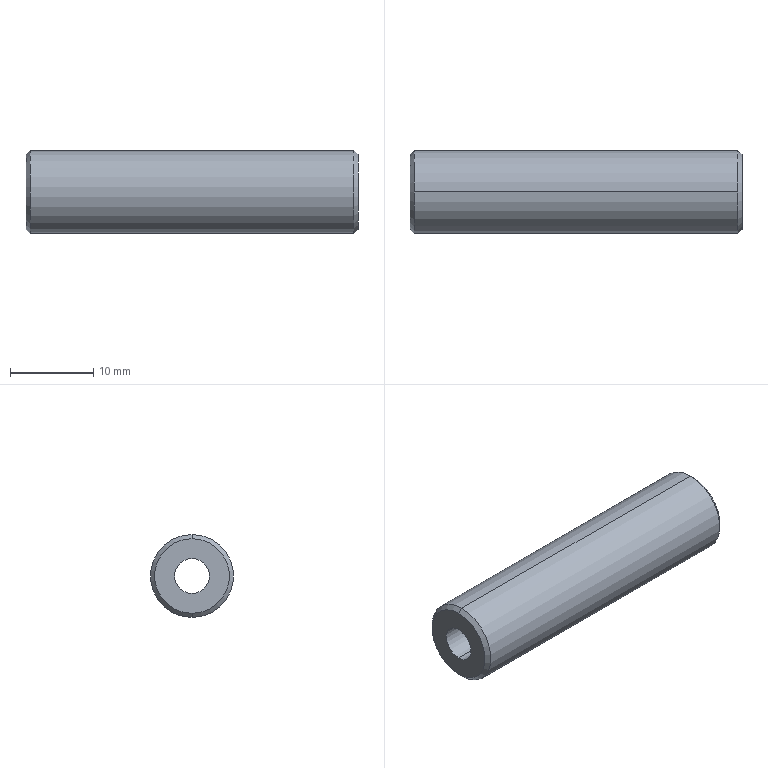Component | SolidWorks | CHEN123-AA-15-2 | 1 solid | 10 faces | box 40 x 10 x 10 mm | volume 2580 mm3 | cone 4 | cylinder 4 | plane 2 | commonest cylinder face diameters 4.2 x2 10 x2
build123d program:
from build123d import *

# Parameters (mm, degrees)
SKETCH1_R           = 5
BOSS_EXTRUDE1_DEPTH = 40
M5_TAPPED_HOLE1_D   = 4.2
CHAMFER1_SIZE       = 0.5


with BuildPart() as part:
    # Sketch1 → Boss-Extrude1 (new body)
    with BuildSketch(Plane.XY):
        Circle(SKETCH1_R)
    extrude(amount=BOSS_EXTRUDE1_DEPTH)

    # M5 Tapped Hole1 (through all)
    with Locations(Plane.XY.offset(40)):
        with Locations((0, 0)):
            Hole(M5_TAPPED_HOLE1_D / 2)

    # Chamfer1
    chamfer1_edges = [part.edges().sort_by_distance(p)[0] for p in [
        (-5, 0, 0),
        (-5, 0, 40),
    ]]
    chamfer(chamfer1_edges, length=CHAMFER1_SIZE)


solid = part.part

# Placed as in the assembly
solid = solid.moved(Location((-20, -132.097, -158.067), (0, 90, 0)))
STEP:
#1=COLOUR_RGB('',0.7922,0.8196,0.9333);
#2=FILL_AREA_STYLE_COLOUR('',#1);
#3=FILL_AREA_STYLE('',(#2));
#4=SURFACE_STYLE_FILL_AREA(#3);
#5=SURFACE_SIDE_STYLE('',(#4));
#6=SURFACE_STYLE_USAGE(.BOTH.,#5);
#7=PRESENTATION_STYLE_ASSIGNMENT((#6));
#8=CARTESIAN_POINT('',(-0.7874,-5.201,-6.046));
#9=VERTEX_POINT('',#8);
#10=CARTESIAN_POINT('',(-0.7874,-5.201,-6.4));
#11=VERTEX_POINT('',#10);
#12=CARTESIAN_POINT('',(-0.7874,-5.201,-6.223));
#13=DIRECTION('',(-1.,0.,0.));
#14=DIRECTION('',(0.,0.,1.));
#15=AXIS2_PLACEMENT_3D('',#12,#13,#14);
#16=CIRCLE('',#15,0.1772);
#17=EDGE_CURVE('',#9,#11,#16,.T.);
#18=ORIENTED_EDGE('',*,*,#17,.F.);
#19=CARTESIAN_POINT('',(-0.7677,-5.201,-6.026));
#20=VERTEX_POINT('',#19);
#21=CARTESIAN_POINT('',(-0.7874,-5.201,-6.046));
#22=DIRECTION('',(0.7071,0.,0.7071));
#23=VECTOR('',#22,39.37);
#24=LINE('',#21,#23);
#25=EDGE_CURVE('',#9,#20,#24,.T.);
#26=ORIENTED_EDGE('',*,*,#25,.T.);
#27=CARTESIAN_POINT('',(-0.7677,-5.201,-6.42));
#28=VERTEX_POINT('',#27);
#29=CARTESIAN_POINT('',(-0.7677,-5.201,-6.223));
#30=DIRECTION('',(1.,0.,0.));
#31=DIRECTION('',(0.,0.,1.));
#32=AXIS2_PLACEMENT_3D('',#29,#30,#31);
#33=CIRCLE('',#32,0.1969);
#34=EDGE_CURVE('',#28,#20,#33,.T.);
#35=ORIENTED_EDGE('',*,*,#34,.F.);
#36=CARTESIAN_POINT('',(-0.7874,-5.201,-6.4));
#37=DIRECTION('',(0.7071,0.,-0.7071));
#38=VECTOR('',#37,39.37);
#39=LINE('',#36,#38);
#40=EDGE_CURVE('',#11,#28,#39,.T.);
#41=ORIENTED_EDGE('',*,*,#40,.F.);
#42=EDGE_LOOP('',(#18,#26,#35,#41));
#43=FACE_OUTER_BOUND('',#42,.T.);
#44=CARTESIAN_POINT('',(-0.7874,-5.201,-6.223));
#45=DIRECTION('',(1.,0.,0.));
#46=DIRECTION('',(0.,0.,-1.));
#47=AXIS2_PLACEMENT_3D('',#44,#45,#46);
#48=CONICAL_SURFACE('',#47,0.1772,0.7854);
#49=ADVANCED_FACE('',(#43),#48,.T.);
#50=CARTESIAN_POINT('',(0.7874,-5.201,-6.4));
#51=VERTEX_POINT('',#50);
#52=CARTESIAN_POINT('',(0.7874,-5.201,-6.046));
#53=VERTEX_POINT('',#52);
#54=CARTESIAN_POINT('',(0.7874,-5.201,-6.223));
#55=DIRECTION('',(1.,0.,0.));
#56=DIRECTION('',(0.,0.,1.));
#57=AXIS2_PLACEMENT_3D('',#54,#55,#56);
#58=CIRCLE('',#57,0.1772);
#59=EDGE_CURVE('',#51,#53,#58,.T.);
#60=ORIENTED_EDGE('',*,*,#59,.F.);
#61=CARTESIAN_POINT('',(0.7677,-5.201,-6.42));
#62=VERTEX_POINT('',#61);
#63=CARTESIAN_POINT('',(0.7677,-5.201,-6.42));
#64=DIRECTION('',(-0.7071,0.,-0.7071));
#65=VECTOR('',#64,39.37);
#66=LINE('',#63,#65);
#67=EDGE_CURVE('',#51,#62,#66,.T.);
#68=ORIENTED_EDGE('',*,*,#67,.T.);
#69=CARTESIAN_POINT('',(0.7677,-5.201,-6.026));
#70=VERTEX_POINT('',#69);
#71=CARTESIAN_POINT('',(0.7677,-5.201,-6.223));
#72=DIRECTION('',(-1.,0.,0.));
#73=DIRECTION('',(0.,0.,1.));
#74=AXIS2_PLACEMENT_3D('',#71,#72,#73);
#75=CIRCLE('',#74,0.1969);
#76=EDGE_CURVE('',#70,#62,#75,.T.);
#77=ORIENTED_EDGE('',*,*,#76,.F.);
#78=CARTESIAN_POINT('',(0.7677,-5.201,-6.026));
#79=DIRECTION('',(-0.7071,0.,0.7071));
#80=VECTOR('',#79,39.37);
#81=LINE('',#78,#80);
#82=EDGE_CURVE('',#53,#70,#81,.T.);
#83=ORIENTED_EDGE('',*,*,#82,.F.);
#84=EDGE_LOOP('',(#60,#68,#77,#83));
#85=FACE_OUTER_BOUND('',#84,.T.);
#86=CARTESIAN_POINT('',(0.7677,-5.201,-6.223));
#87=DIRECTION('',(-1.,0.,0.));
#88=DIRECTION('',(0.,0.,1.));
#89=AXIS2_PLACEMENT_3D('',#86,#87,#88);
#90=CONICAL_SURFACE('',#89,0.1969,0.7854);
#91=ADVANCED_FACE('',(#85),#90,.T.);
#92=CARTESIAN_POINT('',(0.7874,-5.201,-6.306));
#93=VERTEX_POINT('',#92);
#94=CARTESIAN_POINT('',(0.7874,-5.201,-6.14));
#95=VERTEX_POINT('',#94);
#96=CARTESIAN_POINT('',(0.7874,-5.201,-6.223));
#97=DIRECTION('',(-1.,0.,0.));
#98=DIRECTION('',(0.,0.,1.));
#99=AXIS2_PLACEMENT_3D('',#96,#97,#98);
#100=CIRCLE('',#99,0.08268);
#101=EDGE_CURVE('',#93,#95,#100,.T.);
#102=ORIENTED_EDGE('',*,*,#101,.F.);
#103=CARTESIAN_POINT('',(-0.7874,-5.201,-6.306));
#104=VERTEX_POINT('',#103);
#105=CARTESIAN_POINT('',(-0.7874,-5.201,-6.306));
#106=DIRECTION('',(-1.,0.,0.));
#107=VECTOR('',#106,39.37);
#108=LINE('',#105,#107);
#109=EDGE_CURVE('',#93,#104,#108,.T.);
#110=ORIENTED_EDGE('',*,*,#109,.T.);
#111=CARTESIAN_POINT('',(-0.7874,-5.201,-6.14));
#112=VERTEX_POINT('',#111);
#113=CARTESIAN_POINT('',(-0.7874,-5.201,-6.223));
#114=DIRECTION('',(-1.,0.,0.));
#115=DIRECTION('',(0.,0.,1.));
#116=AXIS2_PLACEMENT_3D('',#113,#114,#115);
#117=CIRCLE('',#116,0.08268);
#118=EDGE_CURVE('',#104,#112,#117,.T.);
#119=ORIENTED_EDGE('',*,*,#118,.T.);
#120=CARTESIAN_POINT('',(-0.7874,-5.201,-6.14));
#121=DIRECTION('',(-1.,0.,0.));
#122=VECTOR('',#121,39.37);
#123=LINE('',#120,#122);
#124=EDGE_CURVE('',#95,#112,#123,.T.);
#125=ORIENTED_EDGE('',*,*,#124,.F.);
#126=EDGE_LOOP('',(#102,#110,#119,#125));
#127=FACE_OUTER_BOUND('',#126,.T.);
#128=CARTESIAN_POINT('',(-0.7874,-5.201,-6.223));
#129=DIRECTION('',(-1.,0.,0.));
#130=DIRECTION('',(0.,0.,1.));
#131=AXIS2_PLACEMENT_3D('',#128,#129,#130);
#132=CYLINDRICAL_SURFACE('',#131,0.08268);
#133=ADVANCED_FACE('',(#127),#132,.F.);
#134=ORIENTED_EDGE('',*,*,#34,.T.);
#135=CARTESIAN_POINT('',(-0.7874,-5.201,-6.026));
#136=DIRECTION('',(1.,0.,0.));
#137=VECTOR('',#136,39.37);
#138=LINE('',#135,#137);
#139=EDGE_CURVE('',#20,#70,#138,.T.);
#140=ORIENTED_EDGE('',*,*,#139,.T.);
#141=ORIENTED_EDGE('',*,*,#76,.T.);
#142=CARTESIAN_POINT('',(-0.7874,-5.201,-6.42));
#143=DIRECTION('',(1.,0.,0.));
#144=VECTOR('',#143,39.37);
#145=LINE('',#142,#144);
#146=EDGE_CURVE('',#28,#62,#145,.T.);
#147=ORIENTED_EDGE('',*,*,#146,.F.);
#148=EDGE_LOOP('',(#134,#140,#141,#147));
#149=FACE_OUTER_BOUND('',#148,.T.);
#150=CARTESIAN_POINT('',(-0.7874,-5.201,-6.223));
#151=DIRECTION('',(1.,0.,0.));
#152=DIRECTION('',(0.,0.,-1.));
#153=AXIS2_PLACEMENT_3D('',#150,#151,#152);
#154=CYLINDRICAL_SURFACE('',#153,0.1969);
#155=ADVANCED_FACE('',(#149),#154,.T.);
#156=ORIENTED_EDGE('',*,*,#139,.F.);
#157=CARTESIAN_POINT('',(-0.7677,-5.201,-6.223));
#158=DIRECTION('',(1.,0.,0.));
#159=DIRECTION('',(0.,0.,1.));
#160=AXIS2_PLACEMENT_3D('',#157,#158,#159);
#161=CIRCLE('',#160,0.1969);
#162=EDGE_CURVE('',#20,#28,#161,.T.);
#163=ORIENTED_EDGE('',*,*,#162,.T.);
#164=ORIENTED_EDGE('',*,*,#146,.T.);
#165=CARTESIAN_POINT('',(0.7677,-5.201,-6.223));
#166=DIRECTION('',(-1.,0.,0.));
#167=DIRECTION('',(0.,0.,1.));
#168=AXIS2_PLACEMENT_3D('',#165,#166,#167);
#169=CIRCLE('',#168,0.1969);
#170=EDGE_CURVE('',#62,#70,#169,.T.);
#171=ORIENTED_EDGE('',*,*,#170,.T.);
#172=EDGE_LOOP('',(#156,#163,#164,#171));
#173=FACE_OUTER_BOUND('',#172,.T.);
#174=CARTESIAN_POINT('',(-0.7874,-5.201,-6.223));
#175=DIRECTION('',(1.,0.,0.));
#176=DIRECTION('',(0.,0.,-1.));
#177=AXIS2_PLACEMENT_3D('',#174,#175,#176);
#178=CYLINDRICAL_SURFACE('',#177,0.1969);
#179=ADVANCED_FACE('',(#173),#178,.T.);
#180=CARTESIAN_POINT('',(-0.7874,-5.201,-6.223));
#181=DIRECTION('',(-1.,0.,0.));
#182=DIRECTION('',(0.,0.,1.));
#183=AXIS2_PLACEMENT_3D('',#180,#181,#182);
#184=CIRCLE('',#183,0.1772);
#185=EDGE_CURVE('',#11,#9,#184,.T.);
#186=ORIENTED_EDGE('',*,*,#185,.T.);
#187=ORIENTED_EDGE('',*,*,#17,.T.);
#188=EDGE_LOOP('',(#186,#187));
#189=FACE_OUTER_BOUND('',#188,.T.);
#190=CARTESIAN_POINT('',(-0.7874,-5.201,-6.223));
#191=DIRECTION('',(-1.,0.,0.));
#192=DIRECTION('',(0.,0.,1.));
#193=AXIS2_PLACEMENT_3D('',#190,#191,#192);
#194=CIRCLE('',#193,0.08268);
#195=EDGE_CURVE('',#112,#104,#194,.T.);
#196=ORIENTED_EDGE('',*,*,#195,.F.);
#197=ORIENTED_EDGE('',*,*,#118,.F.);
#198=EDGE_LOOP('',(#196,#197));
#199=FACE_BOUND('',#198,.T.);
#200=CARTESIAN_POINT('',(-0.7874,-5.201,-6.223));
#201=DIRECTION('',(-1.,0.,0.));
#202=DIRECTION('',(0.,0.,1.));
#203=AXIS2_PLACEMENT_3D('',#200,#201,#202);
#204=PLANE('',#203);
#205=ADVANCED_FACE('',(#189,#199),#204,.T.);
#206=CARTESIAN_POINT('',(0.7874,-5.201,-6.223));
#207=DIRECTION('',(1.,0.,0.));
#208=DIRECTION('',(0.,0.,1.));
#209=AXIS2_PLACEMENT_3D('',#206,#207,#208);
#210=CIRCLE('',#209,0.1772);
#211=EDGE_CURVE('',#53,#51,#210,.T.);
#212=ORIENTED_EDGE('',*,*,#211,.T.);
#213=ORIENTED_EDGE('',*,*,#59,.T.);
#214=EDGE_LOOP('',(#212,#213));
#215=FACE_OUTER_BOUND('',#214,.T.);
#216=CARTESIAN_POINT('',(0.7874,-5.201,-6.223));
#217=DIRECTION('',(-1.,0.,0.));
#218=DIRECTION('',(0.,0.,1.));
#219=AXIS2_PLACEMENT_3D('',#216,#217,#218);
#220=CIRCLE('',#219,0.08268);
#221=EDGE_CURVE('',#95,#93,#220,.T.);
#222=ORIENTED_EDGE('',*,*,#221,.T.);
#223=ORIENTED_EDGE('',*,*,#101,.T.);
#224=EDGE_LOOP('',(#222,#223));
#225=FACE_BOUND('',#224,.T.);
#226=CARTESIAN_POINT('',(0.7874,-5.201,-6.223));
#227=DIRECTION('',(-1.,0.,0.));
#228=DIRECTION('',(0.,0.,1.));
#229=AXIS2_PLACEMENT_3D('',#226,#227,#228);
#230=PLANE('',#229);
#231=ADVANCED_FACE('',(#215,#225),#230,.F.);
#232=ORIENTED_EDGE('',*,*,#109,.F.);
#233=ORIENTED_EDGE('',*,*,#221,.F.);
#234=ORIENTED_EDGE('',*,*,#124,.T.);
#235=ORIENTED_EDGE('',*,*,#195,.T.);
#236=EDGE_LOOP('',(#232,#233,#234,#235));
#237=FACE_OUTER_BOUND('',#236,.T.);
#238=CARTESIAN_POINT('',(-0.7874,-5.201,-6.223));
#239=DIRECTION('',(-1.,0.,0.));
#240=DIRECTION('',(0.,0.,1.));
#241=AXIS2_PLACEMENT_3D('',#238,#239,#240);
#242=CYLINDRICAL_SURFACE('',#241,0.08268);
#243=ADVANCED_FACE('',(#237),#242,.F.);
#244=ORIENTED_EDGE('',*,*,#67,.F.);
#245=ORIENTED_EDGE('',*,*,#211,.F.);
#246=ORIENTED_EDGE('',*,*,#82,.T.);
#247=ORIENTED_EDGE('',*,*,#170,.F.);
#248=EDGE_LOOP('',(#244,#245,#246,#247));
#249=FACE_OUTER_BOUND('',#248,.T.);
#250=CARTESIAN_POINT('',(0.7677,-5.201,-6.223));
#251=DIRECTION('',(-1.,0.,0.));
#252=DIRECTION('',(0.,0.,1.));
#253=AXIS2_PLACEMENT_3D('',#250,#251,#252);
#254=CONICAL_SURFACE('',#253,0.1969,0.7854);
#255=ADVANCED_FACE('',(#249),#254,.T.);
#256=ORIENTED_EDGE('',*,*,#25,.F.);
#257=ORIENTED_EDGE('',*,*,#185,.F.);
#258=ORIENTED_EDGE('',*,*,#40,.T.);
#259=ORIENTED_EDGE('',*,*,#162,.F.);
#260=EDGE_LOOP('',(#256,#257,#258,#259));
#261=FACE_OUTER_BOUND('',#260,.T.);
#262=CARTESIAN_POINT('',(-0.7874,-5.201,-6.223));
#263=DIRECTION('',(1.,0.,0.));
#264=DIRECTION('',(0.,0.,-1.));
#265=AXIS2_PLACEMENT_3D('',#262,#263,#264);
#266=CONICAL_SURFACE('',#265,0.1772,0.7854);
#267=ADVANCED_FACE('',(#261),#266,.T.);
#268=CLOSED_SHELL('',(#49,#91,#133,#155,#179,#205,#231,#243,#255,#267));
#269=MANIFOLD_SOLID_BREP('',#268);
#270=STYLED_ITEM('',(#7),#269);
#271=PRESENTATION_LAYER_ASSIGNMENT('','',(#270));
#272=CARTESIAN_POINT('',(0.,0.,0.));
#273=DIRECTION('',(0.,0.,1.));
#274=DIRECTION('',(1.,0.,0.));
#275=AXIS2_PLACEMENT_3D('',#272,#273,#274);
#276=(LENGTH_UNIT()NAMED_UNIT(*)SI_UNIT($,.METRE.));
#277=LENGTH_MEASURE_WITH_UNIT(LENGTH_MEASURE(0.0254),#276);
#278=DIMENSIONAL_EXPONENTS(1.,0.,0.,0.,0.,0.,0.);
#279=(CONVERSION_BASED_UNIT('',#277)LENGTH_UNIT()NAMED_UNIT(#278));
#280=UNCERTAINTY_MEASURE_WITH_UNIT(LENGTH_MEASURE(0.00001),#279,'','');
#281=(NAMED_UNIT(*)PLANE_ANGLE_UNIT()SI_UNIT($,.RADIAN.));
#282=(NAMED_UNIT(*)SI_UNIT($,.STERADIAN.)SOLID_ANGLE_UNIT());
#283=(GEOMETRIC_REPRESENTATION_CONTEXT(3)GLOBAL_UNCERTAINTY_ASSIGNED_CONTEXT((#280))GLOBAL_UNIT_ASSIGNED_CONTEXT((#279,#281,#282))REPRESENTATION_CONTEXT('',''));
#284=ADVANCED_BREP_SHAPE_REPRESENTATION('',(#269,#275),#283);
#285=(LENGTH_UNIT()NAMED_UNIT(*)SI_UNIT($,.METRE.));
#286=LENGTH_MEASURE_WITH_UNIT(LENGTH_MEASURE(0.0254),#285);
#287=DIMENSIONAL_EXPONENTS(1.,0.,0.,0.,0.,0.,0.);
#288=(CONVERSION_BASED_UNIT('',#286)LENGTH_UNIT()NAMED_UNIT(#287));
#289=UNCERTAINTY_MEASURE_WITH_UNIT(LENGTH_MEASURE(0.00001),#288,'','');
#290=(NAMED_UNIT(*)PLANE_ANGLE_UNIT()SI_UNIT($,.RADIAN.));
#291=(NAMED_UNIT(*)SI_UNIT($,.STERADIAN.)SOLID_ANGLE_UNIT());
#292=(GEOMETRIC_REPRESENTATION_CONTEXT(3)GLOBAL_UNCERTAINTY_ASSIGNED_CONTEXT((#289))GLOBAL_UNIT_ASSIGNED_CONTEXT((#288,#290,#291))REPRESENTATION_CONTEXT('',''));
#293=MECHANICAL_DESIGN_GEOMETRIC_PRESENTATION_REPRESENTATION('',(#270),#292);